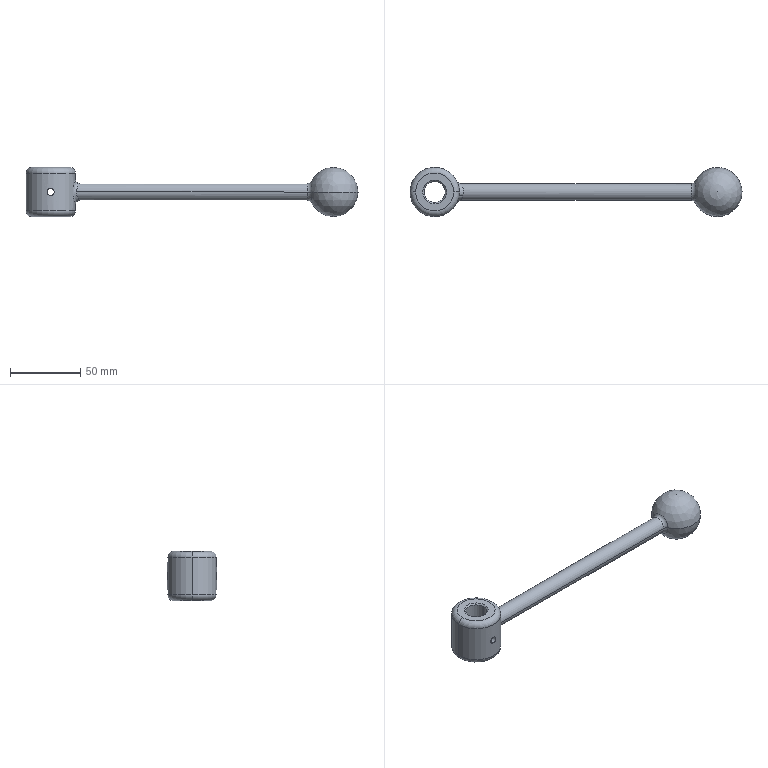Component | SolidWorks | Handle-1 | 1 solid | 26 faces | volume 67717 mm3 | cylinder 10 | torus 6 | cone 4 | spline 2 | sphere 2 | plane 2 | commonest cylinder face diameters 5 x4 15 x2 12 x2 35 x2